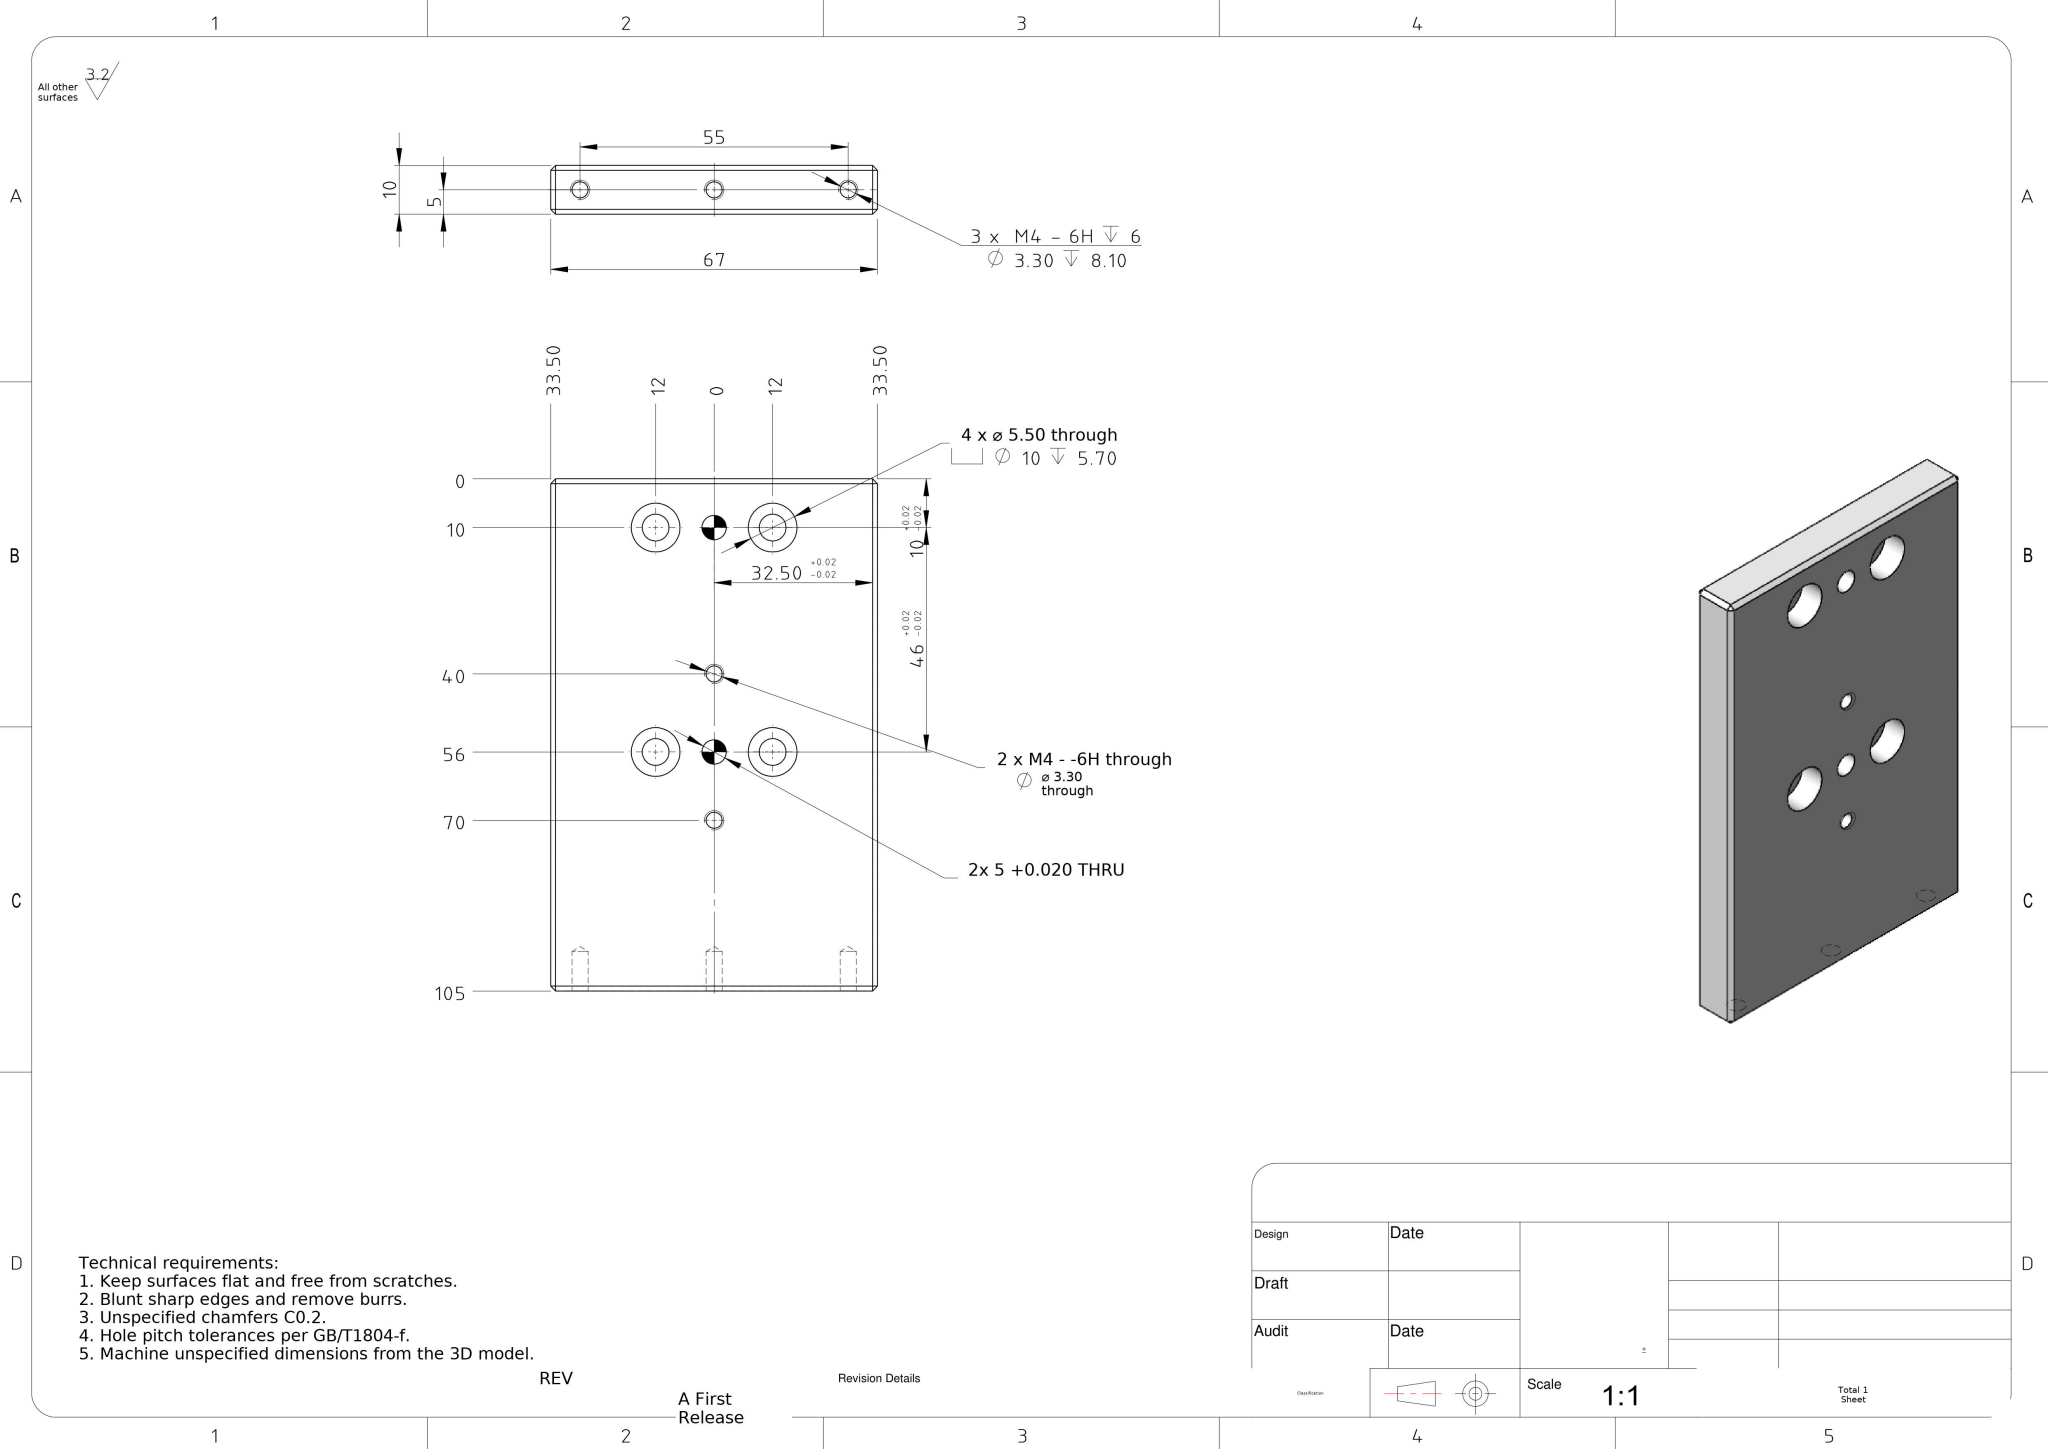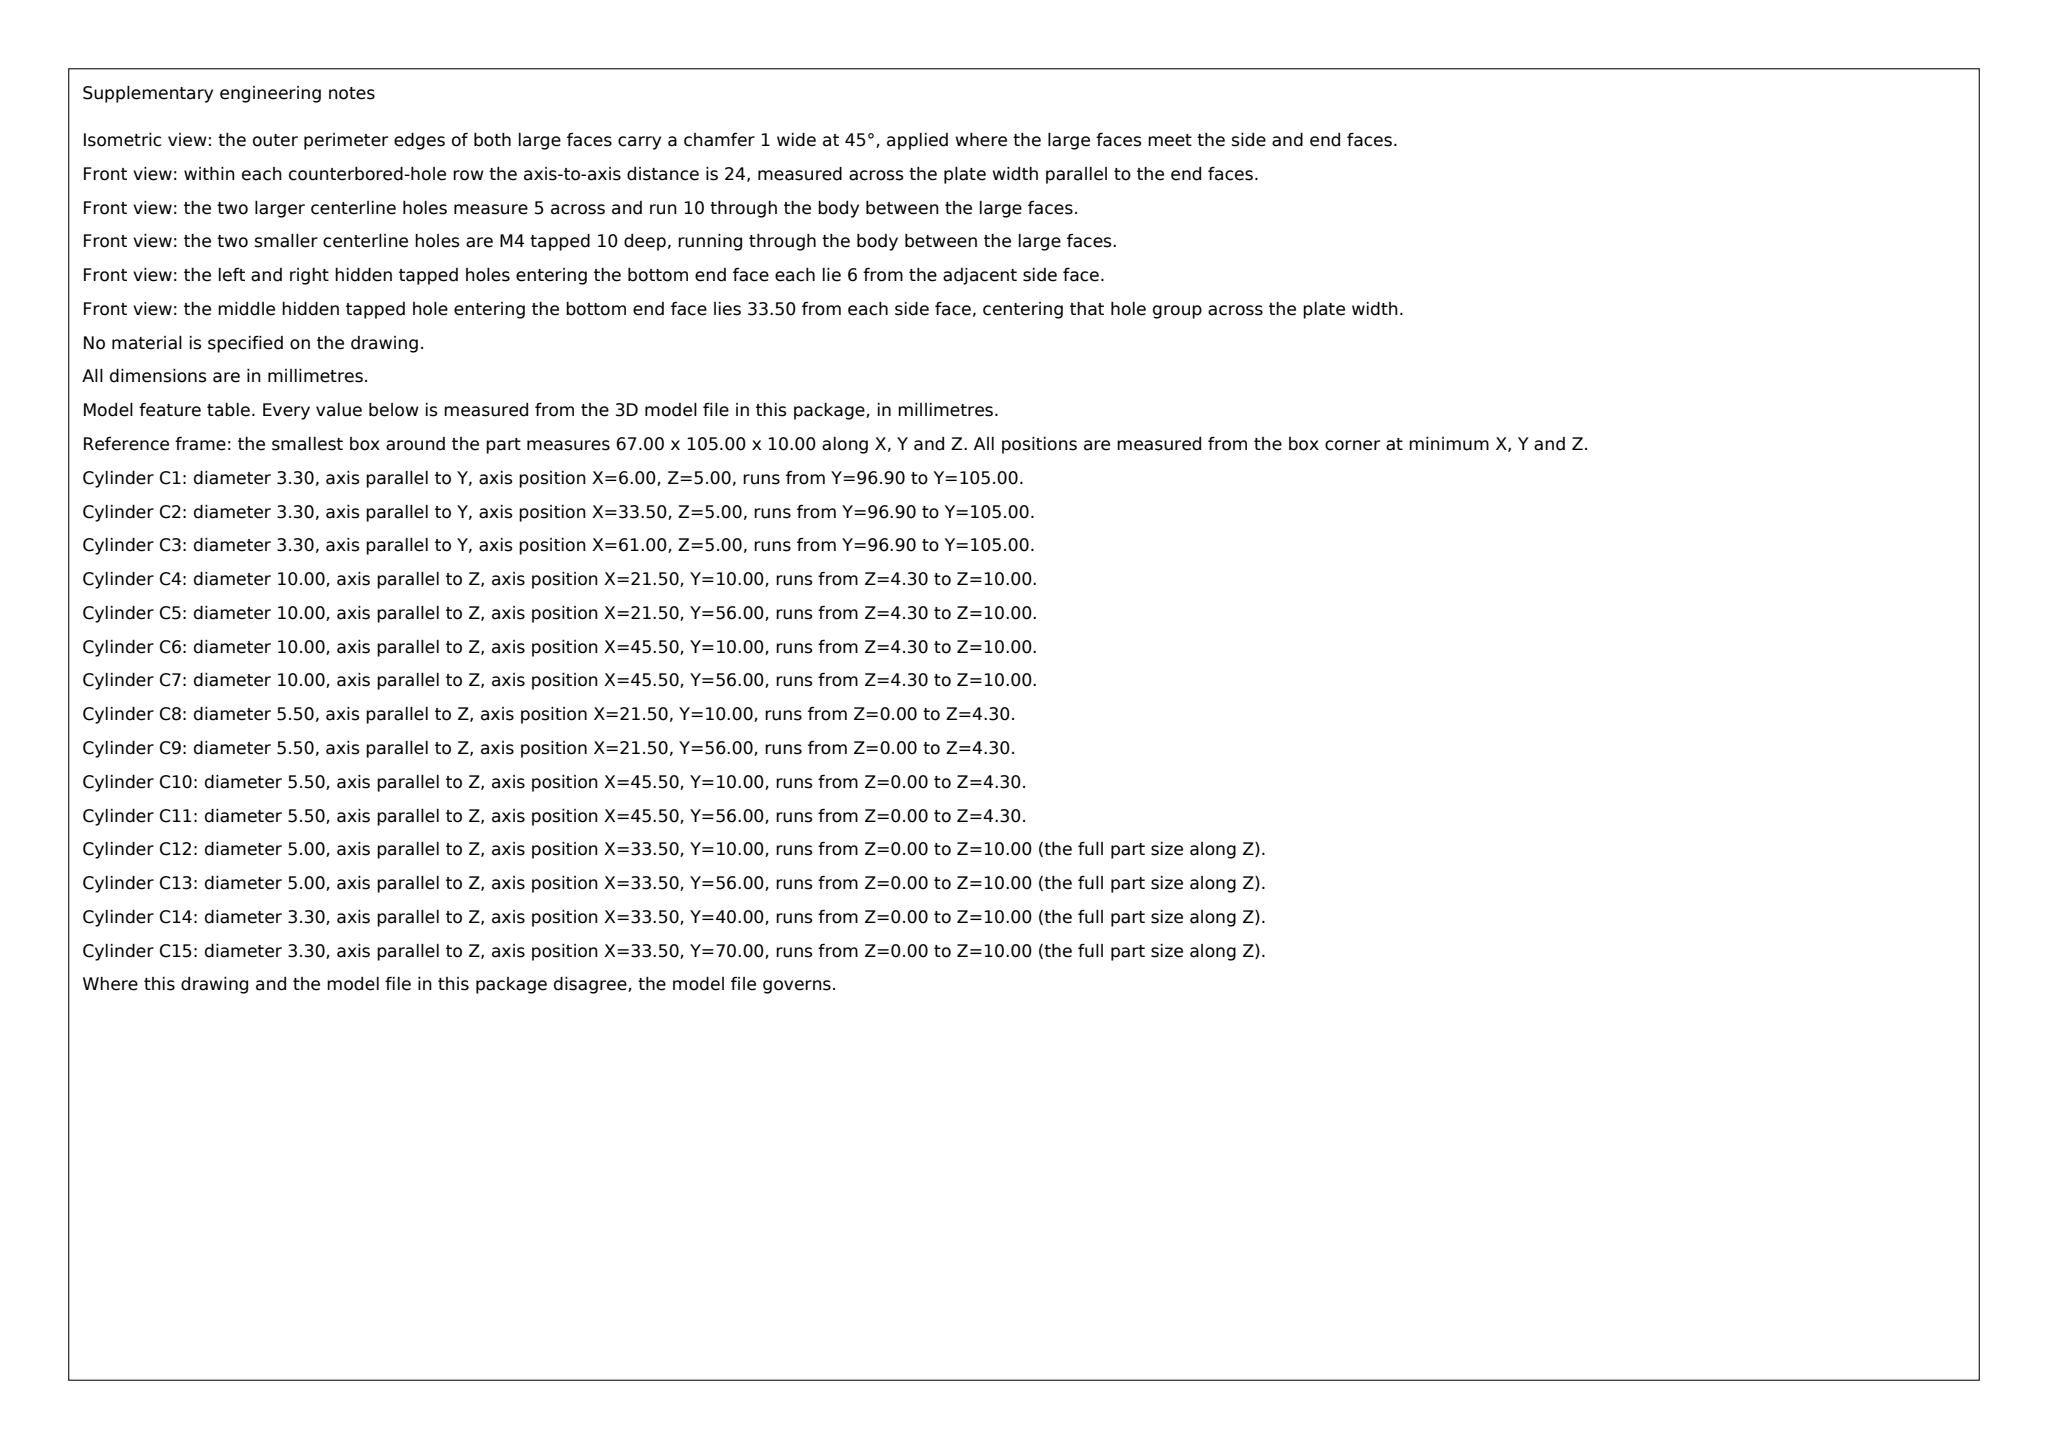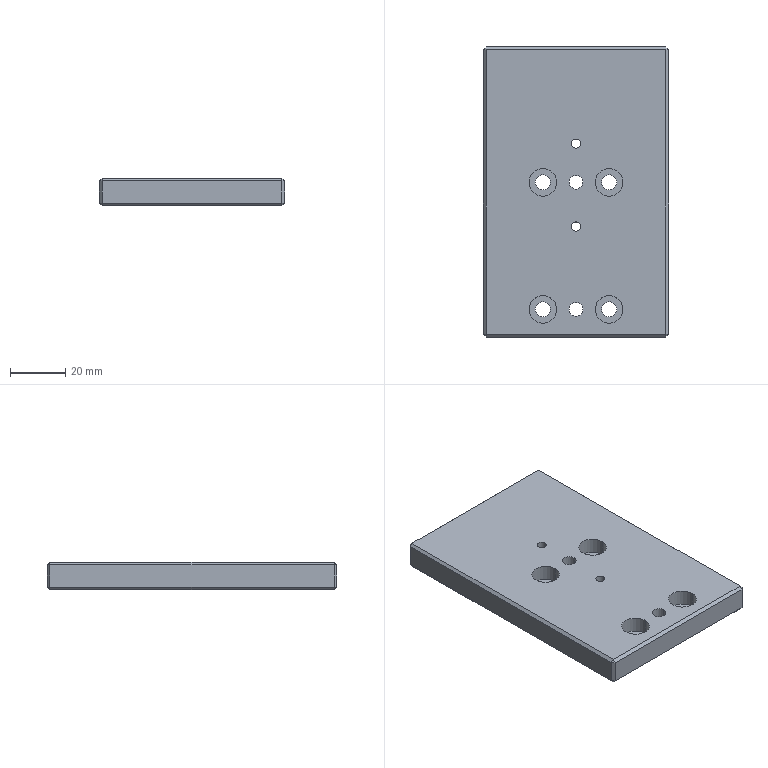Part | SolidWorks | mm | 1 solid | 66 faces | box 67 x 105 x 10 mm | volume 67012 mm3 | cylinder 30 | plane 30 | cone 6 | commonest cylinder face diameters 3.3 x10 10 x8 5.5 x8 5 x4
Drawing notes:
2x Ø5 +0.020/0 THRU, ON CL 12 FROM TOP & 56 FROM TOP | from the solid: cylinders Ø5.0 axis z at (33.5,10) and (33.5,56), from z0 to z10 (THRU 10 thk)
build123d program:
from build123d import *

# Parameters (mm, degrees)
SKETCH1_W                                            = 67
SKETCH1_H                                            = 105
BOSS_EXTRUDE1_DEPTH                                  = 10
HOLE_SIZE_ACCORDING_TO_HEX_SOCKET_HEAD_C_D           = 5.5
HOLE_SIZE_ACCORDING_TO_HEX_SOCKET_HEAD_C_CBORE_D     = 10
HOLE_SIZE_ACCORDING_TO_HEX_SOCKET_HEAD_C_CBORE_DEPTH = 5.7
M4_TAPPED_HOLE1_D                                    = 3.3
M4_TAPPED_HOLE2_D                                    = 3.3
M4_TAPPED_HOLE2_DEPTH                                = 8.1
M4_TAPPED_HOLE2_TIP                                  = 0.9914
SKETCH9_R                                            = 2.5
SKETCH9_R_2                                          = 2.5
CUT_EXTRUDE2_DEPTH                                   = 64.075
CHAMFER1_SIZE                                        = 1


with BuildPart() as part:
    # Sketch1 → Boss-Extrude1 (new body)
    with BuildSketch(Plane.XY):
        Rectangle(SKETCH1_W, SKETCH1_H)
    extrude(amount=BOSS_EXTRUDE1_DEPTH)

    # Hole Size_According to_Hex Socket Head C (through all)
    with Locations(Plane.XY.offset(10)):
        with Locations((12, -42.5), (-12, -42.5), (-12, 3.5), (12, 3.5)):
            CounterBoreHole(HOLE_SIZE_ACCORDING_TO_HEX_SOCKET_HEAD_C_D / 2, HOLE_SIZE_ACCORDING_TO_HEX_SOCKET_HEAD_C_CBORE_D / 2, HOLE_SIZE_ACCORDING_TO_HEX_SOCKET_HEAD_C_CBORE_DEPTH)

    # M4 Tapped Hole1 (through all)
    with Locations(Plane.XY.offset(10)):
        with Locations((0, -12.5), (0, 17.5)):
            Hole(M4_TAPPED_HOLE1_D / 2)

    # M4 Tapped Hole2
    with Locations(Plane(origin=(0, 52.5, 0), x_dir=(1, 0, 0), z_dir=(0, 1, 0))):
        with Locations((27.5, -5), (-27.5, -5), (0, -5)):
            Hole(M4_TAPPED_HOLE2_D / 2, depth=M4_TAPPED_HOLE2_DEPTH)
            with Locations((0, 0, -(M4_TAPPED_HOLE2_DEPTH + M4_TAPPED_HOLE2_TIP / 2))):  # 118° drill point
                Cone(0, M4_TAPPED_HOLE2_D / 2, M4_TAPPED_HOLE2_TIP, mode=Mode.SUBTRACT)

    # Sketch9 → Cut-Extrude2 (cut, through all)
    with BuildSketch(Plane.XY.offset(10)):
        with Locations((0, 3.5)):
            Circle(SKETCH9_R)
        with Locations((0, -42.5)):
            Circle(SKETCH9_R_2)
    extrude(amount=-CUT_EXTRUDE2_DEPTH, mode=Mode.SUBTRACT)

    # Chamfer1
    chamfer1_edges = [part.edges().sort_by_distance(p)[0] for p in [
        (-33.5, 0, 10),
        (0, -52.5, 10),
        (33.5, 0, 10),
        (0, -52.5, 0),
        (-33.5, 0, 0),
        (0, 52.5, 0),
        (33.5, 0, 0),
        (0, 52.5, 10),
        (33.5, -52.5, 5),
        (-33.5, -52.5, 5),
        (-33.5, 52.5, 5),
        (33.5, 52.5, 5),
    ]]
    chamfer(chamfer1_edges, length=CHAMFER1_SIZE)


solid = part.part